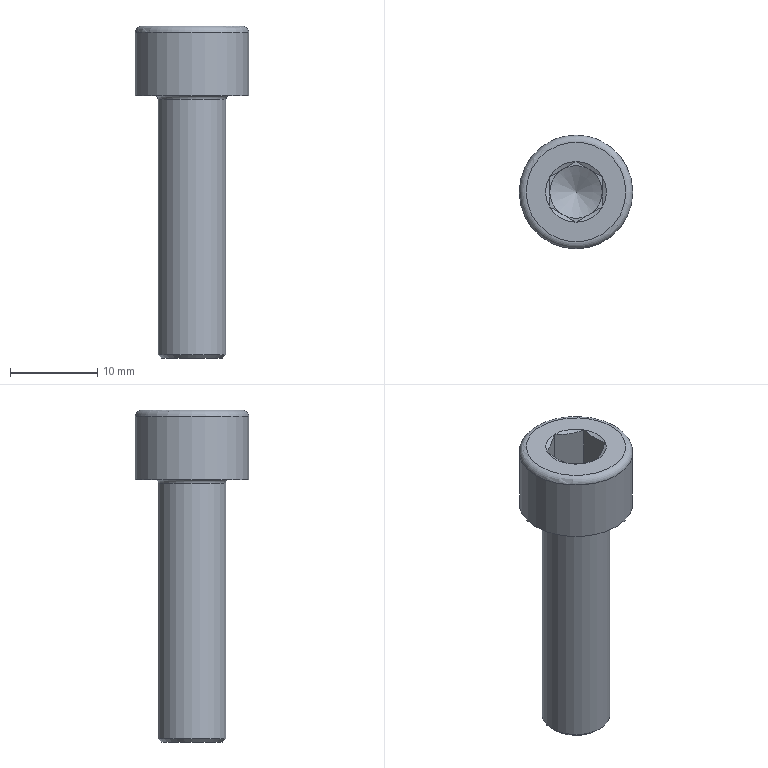Component | NX | GB-T70_1-2000_M8X30 | 1 solid | 27 faces | volume 2310 mm3 | plane 15 | cone 8 | cylinder 2 | torus 2 | commonest cylinder face diameters 7.76 x1 13 x1